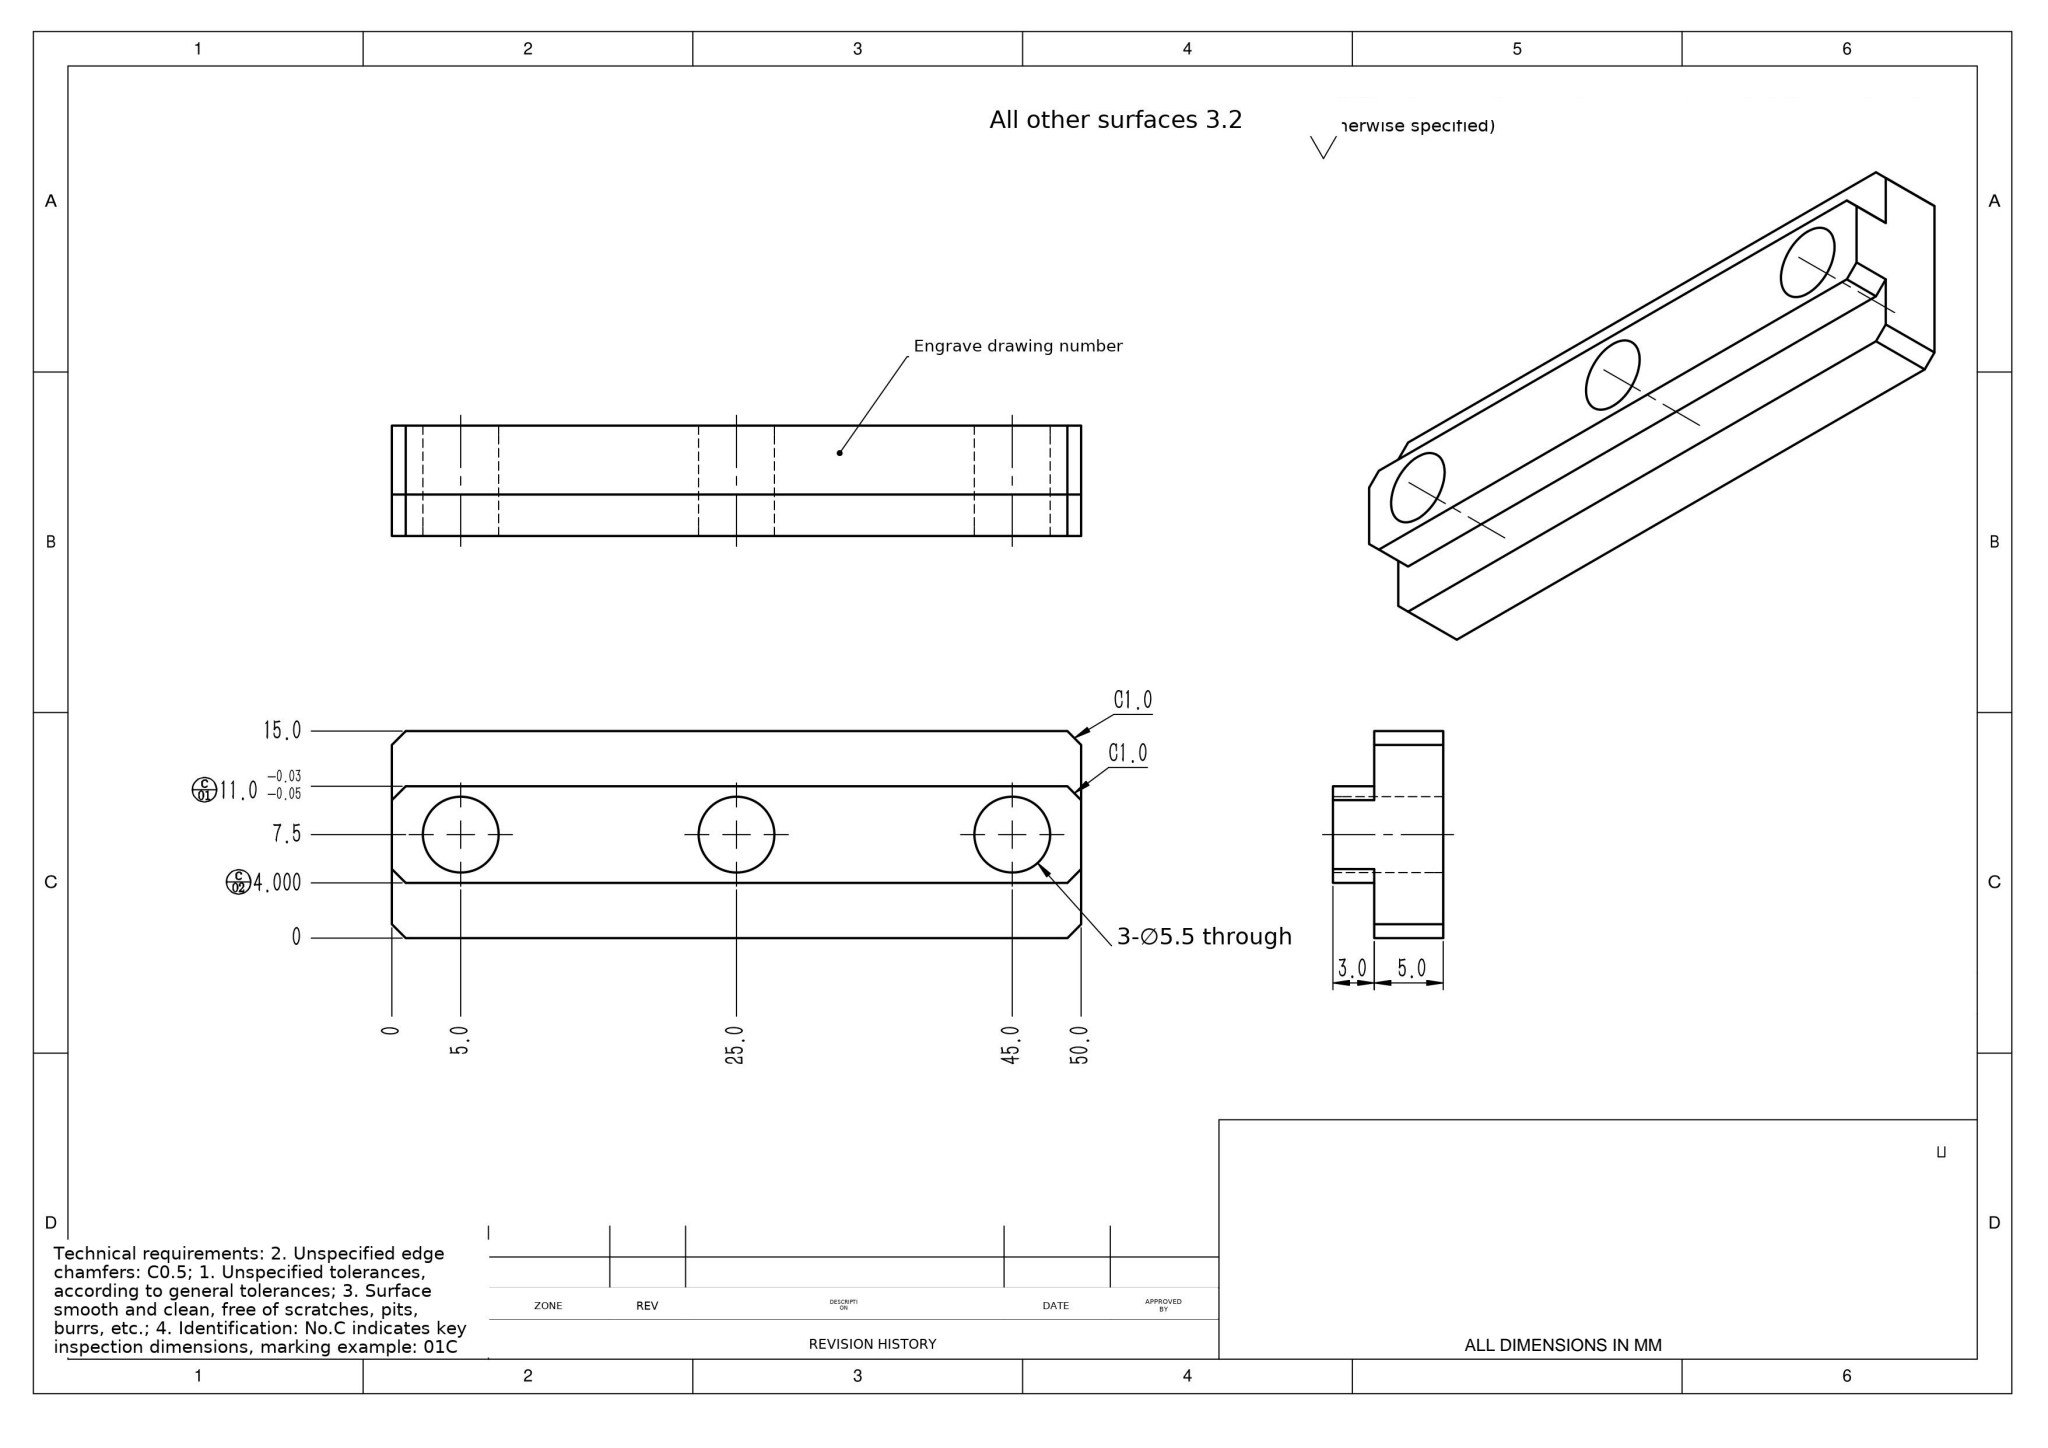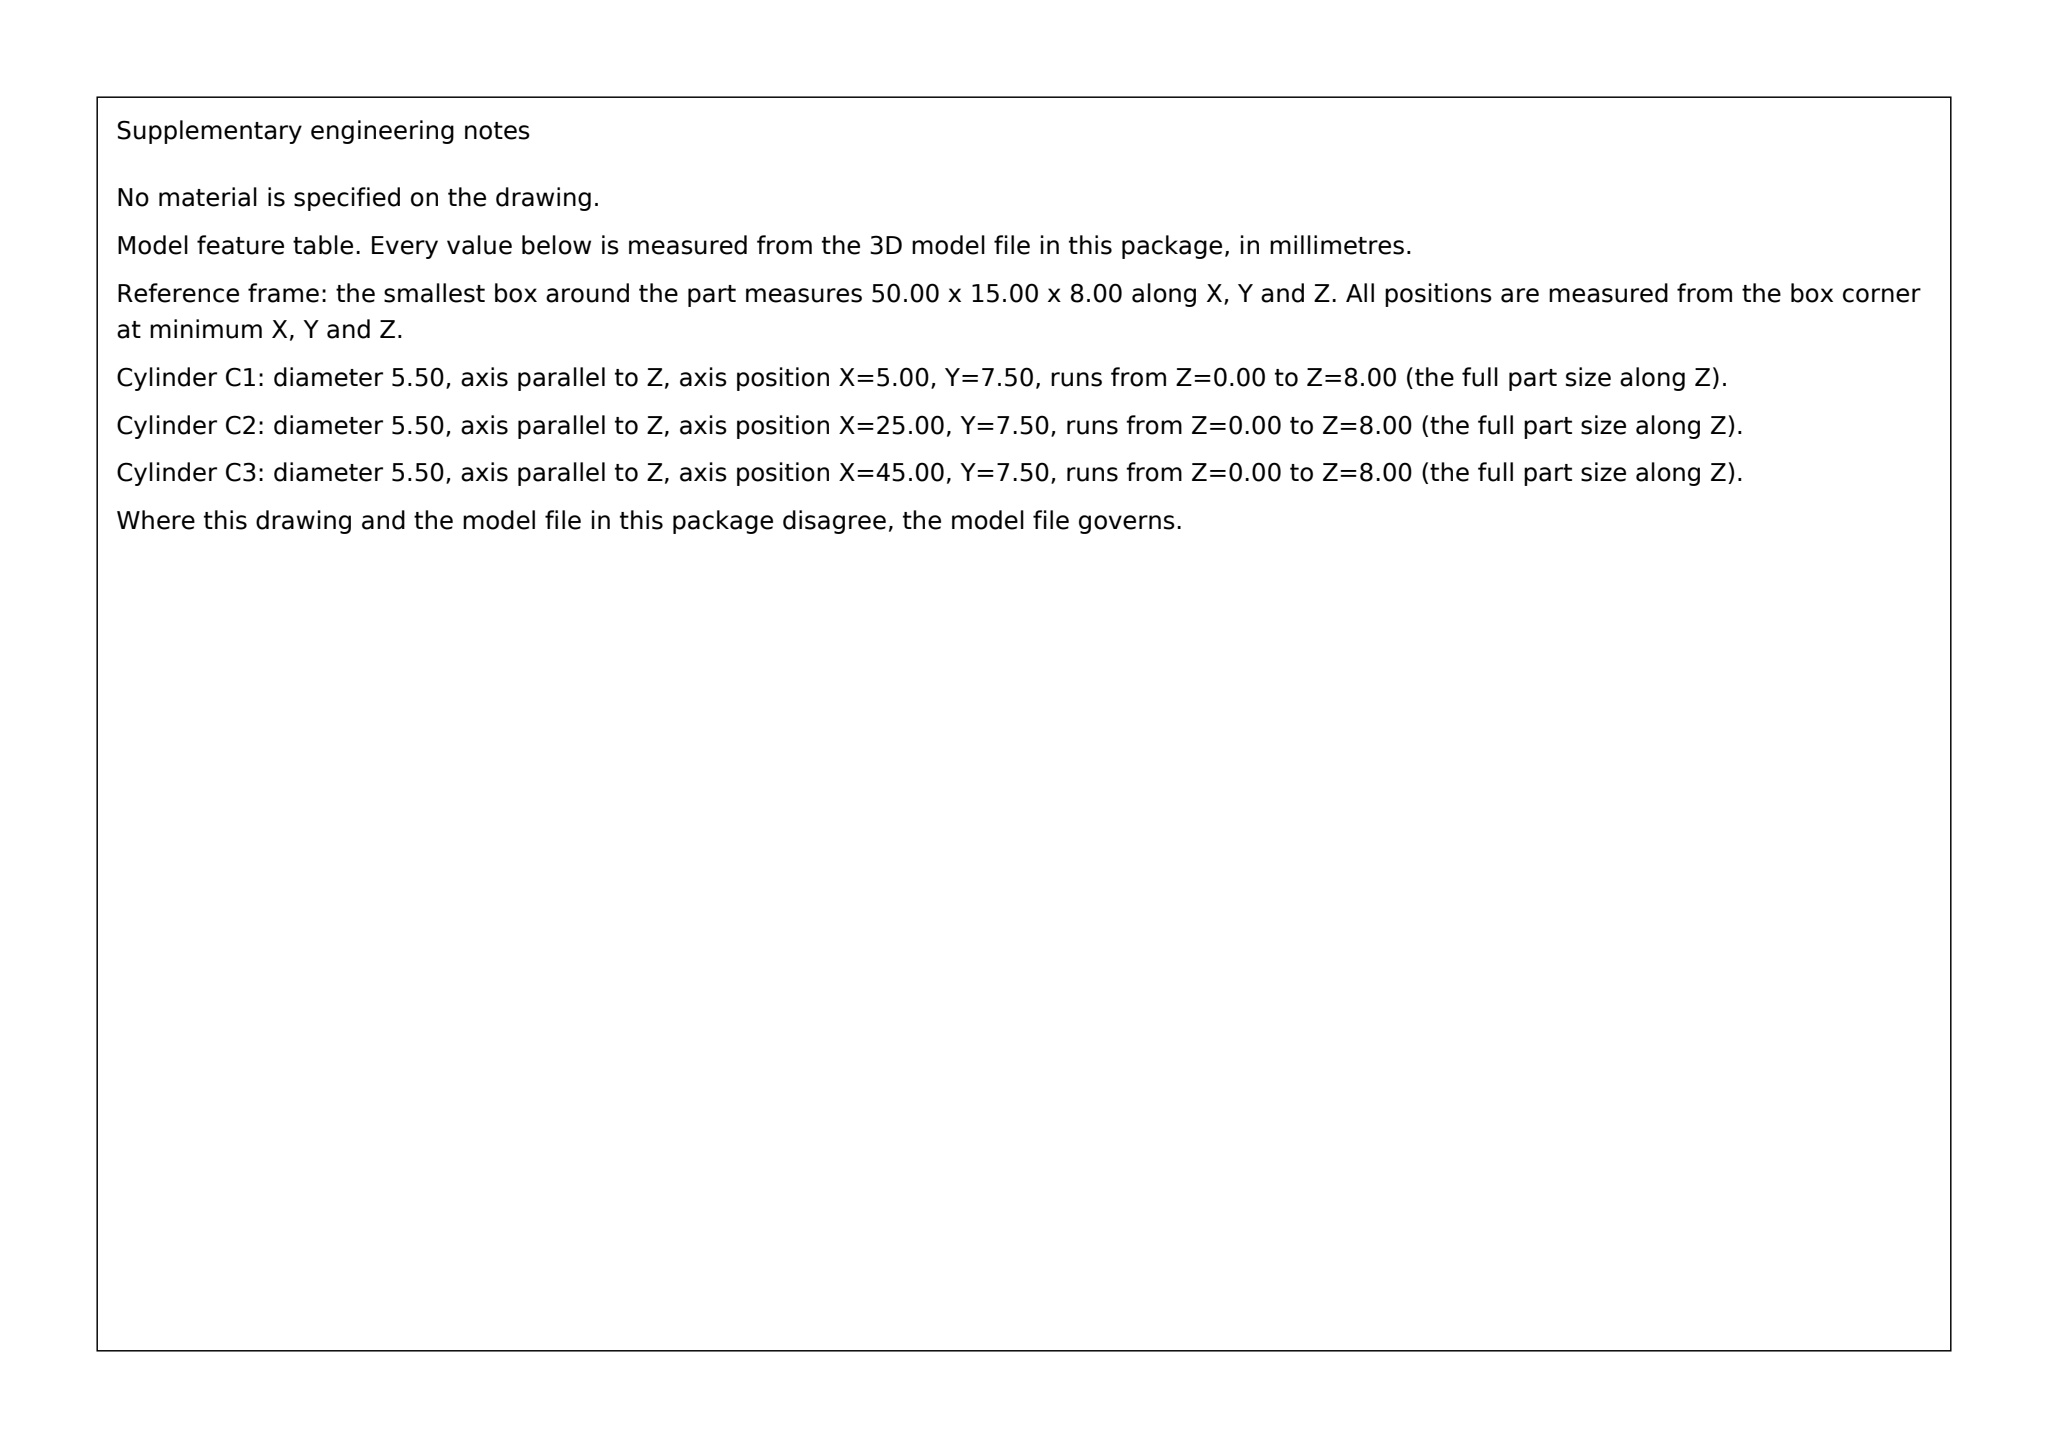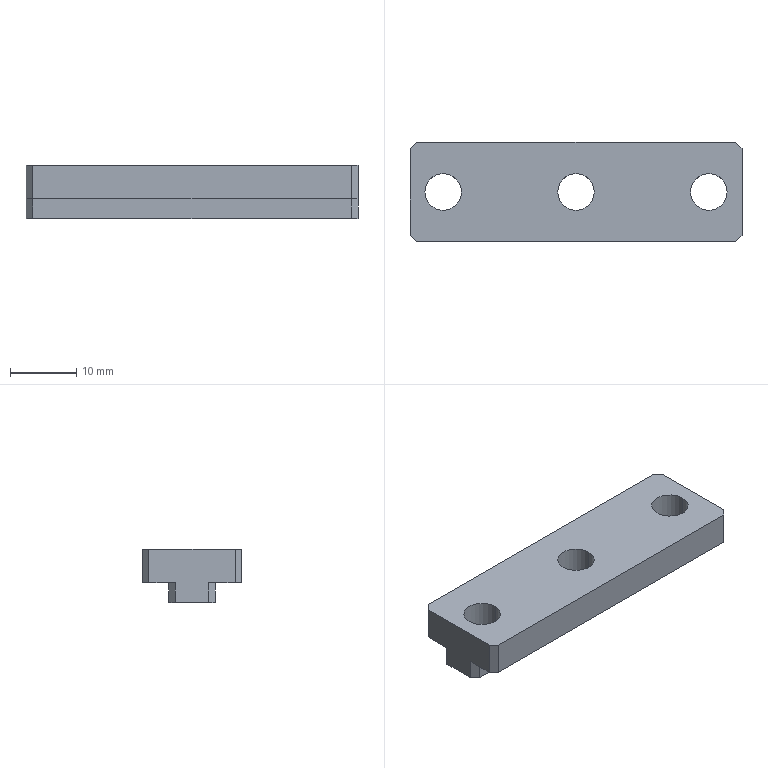Part | SolidWorks | mm | 1 solid | 24 faces | box 50 x 15 x 8 mm | volume 4214 mm3 | plane 18 | cylinder 6 | commonest cylinder face diameters 5.5 x6
build123d program:
from build123d import *

# Parameters (mm, degrees)
SKETCH2_W           = 50
SKETCH2_H           = 7
BOSS_EXTRUDE1_DEPTH = 3
SKETCH3_W           = 50
SKETCH3_H           = 15
BOSS_EXTRUDE2_DEPTH = 5
SKETCH4_R           = 2.75
CUT_EXTRUDE1_DEPTH  = 28.299
CHAMFER1_SIZE       = 1


with BuildPart() as part:
    # Sketch2 → Boss-Extrude1 (new body)
    with BuildSketch(Plane.XY):
        Rectangle(SKETCH2_W, SKETCH2_H)
    extrude(amount=BOSS_EXTRUDE1_DEPTH)

    # Sketch3 → Boss-Extrude2 (add)
    with BuildSketch(Plane.XY.offset(3)):
        Rectangle(SKETCH3_W, SKETCH3_H)
    extrude(amount=BOSS_EXTRUDE2_DEPTH)

    # Sketch4 → Cut-Extrude1 (cut, through all)
    with BuildSketch(Plane.XY.offset(8)):
        Circle(SKETCH4_R)
        with Locations((-20, 0)):
            Circle(SKETCH4_R)
        with Locations((20, 0)):
            Circle(SKETCH4_R)
    extrude(amount=-CUT_EXTRUDE1_DEPTH, mode=Mode.SUBTRACT)

    # Chamfer1
    chamfer1_edges = [part.edges().sort_by_distance(p)[0] for p in [
        (-25, -7.5, 5.5),
        (-25, -3.5, 1.5),
        (-25, 3.5, 1.5),
        (-25, 7.5, 5.5),
        (25, -7.5, 5.5),
        (25, -3.5, 1.5),
        (25, 3.5, 1.5),
        (25, 7.5, 5.5),
    ]]
    chamfer(chamfer1_edges, length=CHAMFER1_SIZE)


solid = part.part
STEP:
#1=CARTESIAN_POINT('',(22.75,0.,0.));
#2=VERTEX_POINT('',#1);
#3=CARTESIAN_POINT('',(17.25,0.,0.));
#4=VERTEX_POINT('',#3);
#5=CARTESIAN_POINT('',(20.,0.,0.));
#6=DIRECTION('',(0.,0.,-1.));
#7=DIRECTION('',(-1.,0.,0.));
#8=AXIS2_PLACEMENT_3D('',#5,#6,#7);
#9=CIRCLE('',#8,2.75);
#10=EDGE_CURVE('',#2,#4,#9,.T.);
#11=ORIENTED_EDGE('',*,*,#10,.T.);
#12=CARTESIAN_POINT('',(17.25,0.,8.));
#13=VERTEX_POINT('',#12);
#14=CARTESIAN_POINT('',(17.25,0.,-0.000025));
#15=DIRECTION('',(0.,0.,1.));
#16=VECTOR('',#15,1000.);
#17=LINE('',#14,#16);
#18=EDGE_CURVE('',#4,#13,#17,.T.);
#19=ORIENTED_EDGE('',*,*,#18,.T.);
#20=CARTESIAN_POINT('',(22.75,0.,8.));
#21=VERTEX_POINT('',#20);
#22=CARTESIAN_POINT('',(20.,0.,8.));
#23=DIRECTION('',(0.,0.,1.));
#24=DIRECTION('',(1.,0.,0.));
#25=AXIS2_PLACEMENT_3D('',#22,#23,#24);
#26=CIRCLE('',#25,2.75);
#27=EDGE_CURVE('',#13,#21,#26,.T.);
#28=ORIENTED_EDGE('',*,*,#27,.T.);
#29=CARTESIAN_POINT('',(22.75,0.,-0.000025));
#30=DIRECTION('',(0.,0.,1.));
#31=VECTOR('',#30,1000.);
#32=LINE('',#29,#31);
#33=EDGE_CURVE('',#2,#21,#32,.T.);
#34=ORIENTED_EDGE('',*,*,#33,.F.);
#35=EDGE_LOOP('',(#11,#19,#28,#34));
#36=FACE_OUTER_BOUND('',#35,.T.);
#37=CARTESIAN_POINT('',(20.,0.,-0.000025));
#38=DIRECTION('',(0.,0.,1.));
#39=DIRECTION('',(1.,0.,0.));
#40=AXIS2_PLACEMENT_3D('',#37,#38,#39);
#41=CYLINDRICAL_SURFACE('',#40,2.75);
#42=ADVANCED_FACE('',(#36),#41,.F.);
#43=CARTESIAN_POINT('',(-17.25,0.,0.));
#44=VERTEX_POINT('',#43);
#45=CARTESIAN_POINT('',(-22.75,0.,0.));
#46=VERTEX_POINT('',#45);
#47=CARTESIAN_POINT('',(-20.,0.,0.));
#48=DIRECTION('',(0.,0.,-1.));
#49=DIRECTION('',(-1.,0.,0.));
#50=AXIS2_PLACEMENT_3D('',#47,#48,#49);
#51=CIRCLE('',#50,2.75);
#52=EDGE_CURVE('',#44,#46,#51,.T.);
#53=ORIENTED_EDGE('',*,*,#52,.T.);
#54=CARTESIAN_POINT('',(-22.75,0.,8.));
#55=VERTEX_POINT('',#54);
#56=CARTESIAN_POINT('',(-22.75,0.,-0.000025));
#57=DIRECTION('',(0.,0.,1.));
#58=VECTOR('',#57,1000.);
#59=LINE('',#56,#58);
#60=EDGE_CURVE('',#46,#55,#59,.T.);
#61=ORIENTED_EDGE('',*,*,#60,.T.);
#62=CARTESIAN_POINT('',(-17.25,0.,8.));
#63=VERTEX_POINT('',#62);
#64=CARTESIAN_POINT('',(-20.,0.,8.));
#65=DIRECTION('',(0.,0.,1.));
#66=DIRECTION('',(1.,0.,0.));
#67=AXIS2_PLACEMENT_3D('',#64,#65,#66);
#68=CIRCLE('',#67,2.75);
#69=EDGE_CURVE('',#55,#63,#68,.T.);
#70=ORIENTED_EDGE('',*,*,#69,.T.);
#71=CARTESIAN_POINT('',(-17.25,0.,-0.000025));
#72=DIRECTION('',(0.,0.,1.));
#73=VECTOR('',#72,1000.);
#74=LINE('',#71,#73);
#75=EDGE_CURVE('',#44,#63,#74,.T.);
#76=ORIENTED_EDGE('',*,*,#75,.F.);
#77=EDGE_LOOP('',(#53,#61,#70,#76));
#78=FACE_OUTER_BOUND('',#77,.T.);
#79=CARTESIAN_POINT('',(-20.,0.,-0.000025));
#80=DIRECTION('',(0.,0.,1.));
#81=DIRECTION('',(1.,0.,0.));
#82=AXIS2_PLACEMENT_3D('',#79,#80,#81);
#83=CYLINDRICAL_SURFACE('',#82,2.75);
#84=ADVANCED_FACE('',(#78),#83,.F.);
#85=CARTESIAN_POINT('',(2.75,0.,0.));
#86=VERTEX_POINT('',#85);
#87=CARTESIAN_POINT('',(-2.75,0.,0.));
#88=VERTEX_POINT('',#87);
#89=CARTESIAN_POINT('',(0.,0.,0.));
#90=DIRECTION('',(0.,0.,-1.));
#91=DIRECTION('',(-1.,0.,0.));
#92=AXIS2_PLACEMENT_3D('',#89,#90,#91);
#93=CIRCLE('',#92,2.75);
#94=EDGE_CURVE('',#86,#88,#93,.T.);
#95=ORIENTED_EDGE('',*,*,#94,.T.);
#96=CARTESIAN_POINT('',(-2.75,0.,8.));
#97=VERTEX_POINT('',#96);
#98=CARTESIAN_POINT('',(-2.75,0.,-0.000025));
#99=DIRECTION('',(0.,0.,1.));
#100=VECTOR('',#99,1000.);
#101=LINE('',#98,#100);
#102=EDGE_CURVE('',#88,#97,#101,.T.);
#103=ORIENTED_EDGE('',*,*,#102,.T.);
#104=CARTESIAN_POINT('',(2.75,0.,8.));
#105=VERTEX_POINT('',#104);
#106=CARTESIAN_POINT('',(0.,0.,8.));
#107=DIRECTION('',(0.,0.,1.));
#108=DIRECTION('',(1.,0.,0.));
#109=AXIS2_PLACEMENT_3D('',#106,#107,#108);
#110=CIRCLE('',#109,2.75);
#111=EDGE_CURVE('',#97,#105,#110,.T.);
#112=ORIENTED_EDGE('',*,*,#111,.T.);
#113=CARTESIAN_POINT('',(2.75,0.,-0.000025));
#114=DIRECTION('',(0.,0.,1.));
#115=VECTOR('',#114,1000.);
#116=LINE('',#113,#115);
#117=EDGE_CURVE('',#86,#105,#116,.T.);
#118=ORIENTED_EDGE('',*,*,#117,.F.);
#119=EDGE_LOOP('',(#95,#103,#112,#118));
#120=FACE_OUTER_BOUND('',#119,.T.);
#121=CARTESIAN_POINT('',(0.,0.,-0.000025));
#122=DIRECTION('',(0.,0.,1.));
#123=DIRECTION('',(1.,0.,0.));
#124=AXIS2_PLACEMENT_3D('',#121,#122,#123);
#125=CYLINDRICAL_SURFACE('',#124,2.75);
#126=ADVANCED_FACE('',(#120),#125,.F.);
#127=CARTESIAN_POINT('',(25.,-6.5,8.));
#128=VERTEX_POINT('',#127);
#129=CARTESIAN_POINT('',(25.,6.5,8.));
#130=VERTEX_POINT('',#129);
#131=CARTESIAN_POINT('',(25.,-7.5,8.));
#132=DIRECTION('',(0.,1.,0.));
#133=VECTOR('',#132,1000.);
#134=LINE('',#131,#133);
#135=EDGE_CURVE('',#128,#130,#134,.T.);
#136=ORIENTED_EDGE('',*,*,#135,.F.);
#137=CARTESIAN_POINT('',(25.,-6.5,3.));
#138=VERTEX_POINT('',#137);
#139=CARTESIAN_POINT('',(25.,-6.5,3.));
#140=DIRECTION('',(0.,0.,-1.));
#141=VECTOR('',#140,1000.);
#142=LINE('',#139,#141);
#143=EDGE_CURVE('',#128,#138,#142,.T.);
#144=ORIENTED_EDGE('',*,*,#143,.T.);
#145=CARTESIAN_POINT('',(25.,-2.5,3.));
#146=VERTEX_POINT('',#145);
#147=CARTESIAN_POINT('',(25.,-7.5,3.));
#148=DIRECTION('',(0.,1.,0.));
#149=VECTOR('',#148,1000.);
#150=LINE('',#147,#149);
#151=EDGE_CURVE('',#138,#146,#150,.T.);
#152=ORIENTED_EDGE('',*,*,#151,.T.);
#153=CARTESIAN_POINT('',(25.,-2.5,0.));
#154=VERTEX_POINT('',#153);
#155=CARTESIAN_POINT('',(25.,-2.5,3.));
#156=DIRECTION('',(0.,0.,-1.));
#157=VECTOR('',#156,1000.);
#158=LINE('',#155,#157);
#159=EDGE_CURVE('',#146,#154,#158,.T.);
#160=ORIENTED_EDGE('',*,*,#159,.T.);
#161=CARTESIAN_POINT('',(25.,2.5,0.));
#162=VERTEX_POINT('',#161);
#163=CARTESIAN_POINT('',(25.,-3.5,0.));
#164=DIRECTION('',(0.,1.,0.));
#165=VECTOR('',#164,1000.);
#166=LINE('',#163,#165);
#167=EDGE_CURVE('',#154,#162,#166,.T.);
#168=ORIENTED_EDGE('',*,*,#167,.T.);
#169=CARTESIAN_POINT('',(25.,2.5,3.));
#170=VERTEX_POINT('',#169);
#171=CARTESIAN_POINT('',(25.,2.5,3.));
#172=DIRECTION('',(0.,0.,1.));
#173=VECTOR('',#172,1000.);
#174=LINE('',#171,#173);
#175=EDGE_CURVE('',#162,#170,#174,.T.);
#176=ORIENTED_EDGE('',*,*,#175,.T.);
#177=CARTESIAN_POINT('',(25.,6.5,3.));
#178=VERTEX_POINT('',#177);
#179=CARTESIAN_POINT('',(25.,-7.5,3.));
#180=DIRECTION('',(0.,1.,0.));
#181=VECTOR('',#180,1000.);
#182=LINE('',#179,#181);
#183=EDGE_CURVE('',#170,#178,#182,.T.);
#184=ORIENTED_EDGE('',*,*,#183,.T.);
#185=CARTESIAN_POINT('',(25.,6.5,3.));
#186=DIRECTION('',(0.,0.,1.));
#187=VECTOR('',#186,1000.);
#188=LINE('',#185,#187);
#189=EDGE_CURVE('',#178,#130,#188,.T.);
#190=ORIENTED_EDGE('',*,*,#189,.T.);
#191=EDGE_LOOP('',(#136,#144,#152,#160,#168,#176,#184,#190));
#192=FACE_OUTER_BOUND('',#191,.T.);
#193=CARTESIAN_POINT('',(25.,-3.5,3.));
#194=DIRECTION('',(-1.,0.,0.));
#195=DIRECTION('',(0.,0.,1.));
#196=AXIS2_PLACEMENT_3D('',#193,#194,#195);
#197=PLANE('',#196);
#198=ADVANCED_FACE('',(#192),#197,.F.);
#199=CARTESIAN_POINT('',(24.,3.5,0.));
#200=VERTEX_POINT('',#199);
#201=CARTESIAN_POINT('',(-24.,3.5,0.));
#202=VERTEX_POINT('',#201);
#203=CARTESIAN_POINT('',(-25.,3.5,0.));
#204=DIRECTION('',(-1.,0.,0.));
#205=VECTOR('',#204,1000.);
#206=LINE('',#203,#205);
#207=EDGE_CURVE('',#200,#202,#206,.T.);
#208=ORIENTED_EDGE('',*,*,#207,.T.);
#209=CARTESIAN_POINT('',(-24.,3.5,3.));
#210=VERTEX_POINT('',#209);
#211=CARTESIAN_POINT('',(-24.,3.5,3.));
#212=DIRECTION('',(0.,0.,1.));
#213=VECTOR('',#212,1000.);
#214=LINE('',#211,#213);
#215=EDGE_CURVE('',#202,#210,#214,.T.);
#216=ORIENTED_EDGE('',*,*,#215,.T.);
#217=CARTESIAN_POINT('',(24.,3.5,3.));
#218=VERTEX_POINT('',#217);
#219=CARTESIAN_POINT('',(-25.,3.5,3.));
#220=DIRECTION('',(-1.,0.,0.));
#221=VECTOR('',#220,1000.);
#222=LINE('',#219,#221);
#223=EDGE_CURVE('',#218,#210,#222,.T.);
#224=ORIENTED_EDGE('',*,*,#223,.F.);
#225=CARTESIAN_POINT('',(24.,3.5,3.));
#226=DIRECTION('',(0.,0.,-1.));
#227=VECTOR('',#226,1000.);
#228=LINE('',#225,#227);
#229=EDGE_CURVE('',#218,#200,#228,.T.);
#230=ORIENTED_EDGE('',*,*,#229,.T.);
#231=EDGE_LOOP('',(#208,#216,#224,#230));
#232=FACE_OUTER_BOUND('',#231,.T.);
#233=CARTESIAN_POINT('',(-25.,3.5,3.));
#234=DIRECTION('',(0.,-1.,0.));
#235=DIRECTION('',(0.,0.,-1.));
#236=AXIS2_PLACEMENT_3D('',#233,#234,#235);
#237=PLANE('',#236);
#238=ADVANCED_FACE('',(#232),#237,.F.);
#239=CARTESIAN_POINT('',(-25.,-2.5,3.));
#240=VERTEX_POINT('',#239);
#241=CARTESIAN_POINT('',(-25.,-6.5,3.));
#242=VERTEX_POINT('',#241);
#243=CARTESIAN_POINT('',(-25.,-7.5,3.));
#244=DIRECTION('',(0.,-1.,0.));
#245=VECTOR('',#244,1000.);
#246=LINE('',#243,#245);
#247=EDGE_CURVE('',#240,#242,#246,.T.);
#248=ORIENTED_EDGE('',*,*,#247,.T.);
#249=CARTESIAN_POINT('',(-25.,-6.5,8.));
#250=VERTEX_POINT('',#249);
#251=CARTESIAN_POINT('',(-25.,-6.5,3.));
#252=DIRECTION('',(0.,0.,1.));
#253=VECTOR('',#252,1000.);
#254=LINE('',#251,#253);
#255=EDGE_CURVE('',#242,#250,#254,.T.);
#256=ORIENTED_EDGE('',*,*,#255,.T.);
#257=CARTESIAN_POINT('',(-25.,6.5,8.));
#258=VERTEX_POINT('',#257);
#259=CARTESIAN_POINT('',(-25.,-7.5,8.));
#260=DIRECTION('',(0.,-1.,0.));
#261=VECTOR('',#260,1000.);
#262=LINE('',#259,#261);
#263=EDGE_CURVE('',#258,#250,#262,.T.);
#264=ORIENTED_EDGE('',*,*,#263,.F.);
#265=CARTESIAN_POINT('',(-25.,6.5,3.));
#266=VERTEX_POINT('',#265);
#267=CARTESIAN_POINT('',(-25.,6.5,3.));
#268=DIRECTION('',(0.,0.,-1.));
#269=VECTOR('',#268,1000.);
#270=LINE('',#267,#269);
#271=EDGE_CURVE('',#258,#266,#270,.T.);
#272=ORIENTED_EDGE('',*,*,#271,.T.);
#273=CARTESIAN_POINT('',(-25.,2.5,3.));
#274=VERTEX_POINT('',#273);
#275=CARTESIAN_POINT('',(-25.,-7.5,3.));
#276=DIRECTION('',(0.,-1.,0.));
#277=VECTOR('',#276,1000.);
#278=LINE('',#275,#277);
#279=EDGE_CURVE('',#266,#274,#278,.T.);
#280=ORIENTED_EDGE('',*,*,#279,.T.);
#281=CARTESIAN_POINT('',(-25.,2.5,0.));
#282=VERTEX_POINT('',#281);
#283=CARTESIAN_POINT('',(-25.,2.5,3.));
#284=DIRECTION('',(0.,0.,-1.));
#285=VECTOR('',#284,1000.);
#286=LINE('',#283,#285);
#287=EDGE_CURVE('',#274,#282,#286,.T.);
#288=ORIENTED_EDGE('',*,*,#287,.T.);
#289=CARTESIAN_POINT('',(-25.,-2.5,0.));
#290=VERTEX_POINT('',#289);
#291=CARTESIAN_POINT('',(-25.,-3.5,0.));
#292=DIRECTION('',(0.,-1.,0.));
#293=VECTOR('',#292,1000.);
#294=LINE('',#291,#293);
#295=EDGE_CURVE('',#282,#290,#294,.T.);
#296=ORIENTED_EDGE('',*,*,#295,.T.);
#297=CARTESIAN_POINT('',(-25.,-2.5,3.));
#298=DIRECTION('',(0.,0.,1.));
#299=VECTOR('',#298,1000.);
#300=LINE('',#297,#299);
#301=EDGE_CURVE('',#290,#240,#300,.T.);
#302=ORIENTED_EDGE('',*,*,#301,.T.);
#303=EDGE_LOOP('',(#248,#256,#264,#272,#280,#288,#296,#302));
#304=FACE_OUTER_BOUND('',#303,.T.);
#305=CARTESIAN_POINT('',(-25.,-3.5,3.));
#306=DIRECTION('',(1.,0.,0.));
#307=DIRECTION('',(0.,0.,-1.));
#308=AXIS2_PLACEMENT_3D('',#305,#306,#307);
#309=PLANE('',#308);
#310=ADVANCED_FACE('',(#304),#309,.F.);
#311=CARTESIAN_POINT('',(-24.,-3.5,3.));
#312=VERTEX_POINT('',#311);
#313=CARTESIAN_POINT('',(24.,-3.5,3.));
#314=VERTEX_POINT('',#313);
#315=CARTESIAN_POINT('',(-25.,-3.5,3.));
#316=DIRECTION('',(1.,0.,0.));
#317=VECTOR('',#316,1000.);
#318=LINE('',#315,#317);
#319=EDGE_CURVE('',#312,#314,#318,.T.);
#320=ORIENTED_EDGE('',*,*,#319,.F.);
#321=CARTESIAN_POINT('',(-24.,-3.5,0.));
#322=VERTEX_POINT('',#321);
#323=CARTESIAN_POINT('',(-24.,-3.5,3.));
#324=DIRECTION('',(0.,0.,-1.));
#325=VECTOR('',#324,1000.);
#326=LINE('',#323,#325);
#327=EDGE_CURVE('',#312,#322,#326,.T.);
#328=ORIENTED_EDGE('',*,*,#327,.T.);
#329=CARTESIAN_POINT('',(24.,-3.5,0.));
#330=VERTEX_POINT('',#329);
#331=CARTESIAN_POINT('',(-25.,-3.5,0.));
#332=DIRECTION('',(1.,0.,0.));
#333=VECTOR('',#332,1000.);
#334=LINE('',#331,#333);
#335=EDGE_CURVE('',#322,#330,#334,.T.);
#336=ORIENTED_EDGE('',*,*,#335,.T.);
#337=CARTESIAN_POINT('',(24.,-3.5,3.));
#338=DIRECTION('',(0.,0.,1.));
#339=VECTOR('',#338,1000.);
#340=LINE('',#337,#339);
#341=EDGE_CURVE('',#330,#314,#340,.T.);
#342=ORIENTED_EDGE('',*,*,#341,.T.);
#343=EDGE_LOOP('',(#320,#328,#336,#342));
#344=FACE_OUTER_BOUND('',#343,.T.);
#345=CARTESIAN_POINT('',(-25.,-3.5,3.));
#346=DIRECTION('',(0.,1.,0.));
#347=DIRECTION('',(0.,0.,1.));
#348=AXIS2_PLACEMENT_3D('',#345,#346,#347);
#349=PLANE('',#348);
#350=ADVANCED_FACE('',(#344),#349,.F.);
#351=ORIENTED_EDGE('',*,*,#10,.F.);
#352=CARTESIAN_POINT('',(20.,0.,0.));
#353=DIRECTION('',(0.,0.,-1.));
#354=DIRECTION('',(-1.,0.,0.));
#355=AXIS2_PLACEMENT_3D('',#352,#353,#354);
#356=CIRCLE('',#355,2.75);
#357=EDGE_CURVE('',#4,#2,#356,.T.);
#358=ORIENTED_EDGE('',*,*,#357,.F.);
#359=EDGE_LOOP('',(#351,#358));
#360=FACE_BOUND('',#359,.T.);
#361=ORIENTED_EDGE('',*,*,#52,.F.);
#362=CARTESIAN_POINT('',(-20.,0.,0.));
#363=DIRECTION('',(0.,0.,-1.));
#364=DIRECTION('',(-1.,0.,0.));
#365=AXIS2_PLACEMENT_3D('',#362,#363,#364);
#366=CIRCLE('',#365,2.75);
#367=EDGE_CURVE('',#46,#44,#366,.T.);
#368=ORIENTED_EDGE('',*,*,#367,.F.);
#369=EDGE_LOOP('',(#361,#368));
#370=FACE_BOUND('',#369,.T.);
#371=ORIENTED_EDGE('',*,*,#94,.F.);
#372=CARTESIAN_POINT('',(0.,0.,0.));
#373=DIRECTION('',(0.,0.,-1.));
#374=DIRECTION('',(-1.,0.,0.));
#375=AXIS2_PLACEMENT_3D('',#372,#373,#374);
#376=CIRCLE('',#375,2.75);
#377=EDGE_CURVE('',#88,#86,#376,.T.);
#378=ORIENTED_EDGE('',*,*,#377,.F.);
#379=EDGE_LOOP('',(#371,#378));
#380=FACE_BOUND('',#379,.T.);
#381=ORIENTED_EDGE('',*,*,#335,.F.);
#382=CARTESIAN_POINT('',(-13.75,-13.75,0.));
#383=DIRECTION('',(-0.7071,0.7071,0.));
#384=VECTOR('',#383,1000.);
#385=LINE('',#382,#384);
#386=EDGE_CURVE('',#322,#290,#385,.T.);
#387=ORIENTED_EDGE('',*,*,#386,.T.);
#388=ORIENTED_EDGE('',*,*,#295,.F.);
#389=CARTESIAN_POINT('',(-13.75,13.75,0.));
#390=DIRECTION('',(0.7071,0.7071,0.));
#391=VECTOR('',#390,1000.);
#392=LINE('',#389,#391);
#393=EDGE_CURVE('',#282,#202,#392,.T.);
#394=ORIENTED_EDGE('',*,*,#393,.T.);
#395=ORIENTED_EDGE('',*,*,#207,.F.);
#396=CARTESIAN_POINT('',(13.75,13.75,0.));
#397=DIRECTION('',(0.7071,-0.7071,0.));
#398=VECTOR('',#397,1000.);
#399=LINE('',#396,#398);
#400=EDGE_CURVE('',#200,#162,#399,.T.);
#401=ORIENTED_EDGE('',*,*,#400,.T.);
#402=ORIENTED_EDGE('',*,*,#167,.F.);
#403=CARTESIAN_POINT('',(13.75,-13.75,0.));
#404=DIRECTION('',(-0.7071,-0.7071,0.));
#405=VECTOR('',#404,1000.);
#406=LINE('',#403,#405);
#407=EDGE_CURVE('',#154,#330,#406,.T.);
#408=ORIENTED_EDGE('',*,*,#407,.T.);
#409=EDGE_LOOP('',(#381,#387,#388,#394,#395,#401,#402,#408));
#410=FACE_OUTER_BOUND('',#409,.T.);
#411=CARTESIAN_POINT('',(0.,0.,0.));
#412=DIRECTION('',(0.,0.,-1.));
#413=DIRECTION('',(-1.,0.,0.));
#414=AXIS2_PLACEMENT_3D('',#411,#412,#413);
#415=PLANE('',#414);
#416=ADVANCED_FACE('',(#360,#370,#380,#410),#415,.T.);
#417=ORIENTED_EDGE('',*,*,#279,.F.);
#418=CARTESIAN_POINT('',(-24.,7.5,3.));
#419=VERTEX_POINT('',#418);
#420=CARTESIAN_POINT('',(-15.75,15.75,3.));
#421=DIRECTION('',(0.7071,0.7071,0.));
#422=VECTOR('',#421,1000.);
#423=LINE('',#420,#422);
#424=EDGE_CURVE('',#266,#419,#423,.T.);
#425=ORIENTED_EDGE('',*,*,#424,.T.);
#426=CARTESIAN_POINT('',(24.,7.5,3.));
#427=VERTEX_POINT('',#426);
#428=CARTESIAN_POINT('',(-25.,7.5,3.));
#429=DIRECTION('',(-1.,0.,0.));
#430=VECTOR('',#429,1000.);
#431=LINE('',#428,#430);
#432=EDGE_CURVE('',#427,#419,#431,.T.);
#433=ORIENTED_EDGE('',*,*,#432,.F.);
#434=CARTESIAN_POINT('',(15.75,15.75,3.));
#435=DIRECTION('',(0.7071,-0.7071,0.));
#436=VECTOR('',#435,1000.);
#437=LINE('',#434,#436);
#438=EDGE_CURVE('',#427,#178,#437,.T.);
#439=ORIENTED_EDGE('',*,*,#438,.T.);
#440=ORIENTED_EDGE('',*,*,#183,.F.);
#441=CARTESIAN_POINT('',(24.,3.5,3.));
#442=DIRECTION('',(-0.7071,0.7071,0.));
#443=VECTOR('',#442,1000.);
#444=LINE('',#441,#443);
#445=EDGE_CURVE('',#170,#218,#444,.T.);
#446=ORIENTED_EDGE('',*,*,#445,.T.);
#447=ORIENTED_EDGE('',*,*,#223,.T.);
#448=CARTESIAN_POINT('',(-25.,2.5,3.));
#449=DIRECTION('',(-0.7071,-0.7071,0.));
#450=VECTOR('',#449,1000.);
#451=LINE('',#448,#450);
#452=EDGE_CURVE('',#210,#274,#451,.T.);
#453=ORIENTED_EDGE('',*,*,#452,.T.);
#454=EDGE_LOOP('',(#417,#425,#433,#439,#440,#446,#447,#453));
#455=FACE_OUTER_BOUND('',#454,.T.);
#456=CARTESIAN_POINT('',(0.,0.,3.));
#457=DIRECTION('',(0.,0.,-1.));
#458=DIRECTION('',(-1.,0.,0.));
#459=AXIS2_PLACEMENT_3D('',#456,#457,#458);
#460=PLANE('',#459);
#461=ADVANCED_FACE('',(#455),#460,.T.);
#462=ORIENTED_EDGE('',*,*,#432,.T.);
#463=CARTESIAN_POINT('',(-24.,7.5,8.));
#464=VERTEX_POINT('',#463);
#465=CARTESIAN_POINT('',(-24.,7.5,8.));
#466=DIRECTION('',(0.,0.,1.));
#467=VECTOR('',#466,1000.);
#468=LINE('',#465,#467);
#469=EDGE_CURVE('',#419,#464,#468,.T.);
#470=ORIENTED_EDGE('',*,*,#469,.T.);
#471=CARTESIAN_POINT('',(24.,7.5,8.));
#472=VERTEX_POINT('',#471);
#473=CARTESIAN_POINT('',(-25.,7.5,8.));
#474=DIRECTION('',(-1.,0.,0.));
#475=VECTOR('',#474,1000.);
#476=LINE('',#473,#475);
#477=EDGE_CURVE('',#472,#464,#476,.T.);
#478=ORIENTED_EDGE('',*,*,#477,.F.);
#479=CARTESIAN_POINT('',(24.,7.5,8.));
#480=DIRECTION('',(0.,0.,-1.));
#481=VECTOR('',#480,1000.);
#482=LINE('',#479,#481);
#483=EDGE_CURVE('',#472,#427,#482,.T.);
#484=ORIENTED_EDGE('',*,*,#483,.T.);
#485=EDGE_LOOP('',(#462,#470,#478,#484));
#486=FACE_OUTER_BOUND('',#485,.T.);
#487=CARTESIAN_POINT('',(-25.,7.5,8.));
#488=DIRECTION('',(0.,-1.,0.));
#489=DIRECTION('',(0.,0.,-1.));
#490=AXIS2_PLACEMENT_3D('',#487,#488,#489);
#491=PLANE('',#490);
#492=ADVANCED_FACE('',(#486),#491,.F.);
#493=CARTESIAN_POINT('',(-24.,-7.5,8.));
#494=VERTEX_POINT('',#493);
#495=CARTESIAN_POINT('',(24.,-7.5,8.));
#496=VERTEX_POINT('',#495);
#497=CARTESIAN_POINT('',(-25.,-7.5,8.));
#498=DIRECTION('',(1.,0.,0.));
#499=VECTOR('',#498,1000.);
#500=LINE('',#497,#499);
#501=EDGE_CURVE('',#494,#496,#500,.T.);
#502=ORIENTED_EDGE('',*,*,#501,.F.);
#503=CARTESIAN_POINT('',(-24.,-7.5,3.));
#504=VERTEX_POINT('',#503);
#505=CARTESIAN_POINT('',(-24.,-7.5,8.));
#506=DIRECTION('',(0.,0.,-1.));
#507=VECTOR('',#506,1000.);
#508=LINE('',#505,#507);
#509=EDGE_CURVE('',#494,#504,#508,.T.);
#510=ORIENTED_EDGE('',*,*,#509,.T.);
#511=CARTESIAN_POINT('',(24.,-7.5,3.));
#512=VERTEX_POINT('',#511);
#513=CARTESIAN_POINT('',(-25.,-7.5,3.));
#514=DIRECTION('',(1.,0.,0.));
#515=VECTOR('',#514,1000.);
#516=LINE('',#513,#515);
#517=EDGE_CURVE('',#504,#512,#516,.T.);
#518=ORIENTED_EDGE('',*,*,#517,.T.);
#519=CARTESIAN_POINT('',(24.,-7.5,8.));
#520=DIRECTION('',(0.,0.,1.));
#521=VECTOR('',#520,1000.);
#522=LINE('',#519,#521);
#523=EDGE_CURVE('',#512,#496,#522,.T.);
#524=ORIENTED_EDGE('',*,*,#523,.T.);
#525=EDGE_LOOP('',(#502,#510,#518,#524));
#526=FACE_OUTER_BOUND('',#525,.T.);
#527=CARTESIAN_POINT('',(-25.,-7.5,8.));
#528=DIRECTION('',(0.,1.,0.));
#529=DIRECTION('',(0.,0.,1.));
#530=AXIS2_PLACEMENT_3D('',#527,#528,#529);
#531=PLANE('',#530);
#532=ADVANCED_FACE('',(#526),#531,.F.);
#533=CARTESIAN_POINT('',(20.,0.,8.));
#534=DIRECTION('',(0.,0.,1.));
#535=DIRECTION('',(1.,0.,0.));
#536=AXIS2_PLACEMENT_3D('',#533,#534,#535);
#537=CIRCLE('',#536,2.75);
#538=EDGE_CURVE('',#21,#13,#537,.T.);
#539=ORIENTED_EDGE('',*,*,#538,.F.);
#540=ORIENTED_EDGE('',*,*,#27,.F.);
#541=EDGE_LOOP('',(#539,#540));
#542=FACE_BOUND('',#541,.T.);
#543=CARTESIAN_POINT('',(-20.,0.,8.));
#544=DIRECTION('',(0.,0.,1.));
#545=DIRECTION('',(1.,0.,0.));
#546=AXIS2_PLACEMENT_3D('',#543,#544,#545);
#547=CIRCLE('',#546,2.75);
#548=EDGE_CURVE('',#63,#55,#547,.T.);
#549=ORIENTED_EDGE('',*,*,#548,.F.);
#550=ORIENTED_EDGE('',*,*,#69,.F.);
#551=EDGE_LOOP('',(#549,#550));
#552=FACE_BOUND('',#551,.T.);
#553=CARTESIAN_POINT('',(0.,0.,8.));
#554=DIRECTION('',(0.,0.,1.));
#555=DIRECTION('',(1.,0.,0.));
#556=AXIS2_PLACEMENT_3D('',#553,#554,#555);
#557=CIRCLE('',#556,2.75);
#558=EDGE_CURVE('',#105,#97,#557,.T.);
#559=ORIENTED_EDGE('',*,*,#558,.F.);
#560=ORIENTED_EDGE('',*,*,#111,.F.);
#561=EDGE_LOOP('',(#559,#560));
#562=FACE_BOUND('',#561,.T.);
#563=ORIENTED_EDGE('',*,*,#263,.T.);
#564=CARTESIAN_POINT('',(-24.,-7.5,8.));
#565=DIRECTION('',(0.7071,-0.7071,0.));
#566=VECTOR('',#565,1000.);
#567=LINE('',#564,#566);
#568=EDGE_CURVE('',#250,#494,#567,.T.);
#569=ORIENTED_EDGE('',*,*,#568,.T.);
#570=ORIENTED_EDGE('',*,*,#501,.T.);
#571=CARTESIAN_POINT('',(25.,-6.5,8.));
#572=DIRECTION('',(0.7071,0.7071,0.));
#573=VECTOR('',#572,1000.);
#574=LINE('',#571,#573);
#575=EDGE_CURVE('',#496,#128,#574,.T.);
#576=ORIENTED_EDGE('',*,*,#575,.T.);
#577=ORIENTED_EDGE('',*,*,#135,.T.);
#578=CARTESIAN_POINT('',(24.,7.5,8.));
#579=DIRECTION('',(-0.7071,0.7071,0.));
#580=VECTOR('',#579,1000.);
#581=LINE('',#578,#580);
#582=EDGE_CURVE('',#130,#472,#581,.T.);
#583=ORIENTED_EDGE('',*,*,#582,.T.);
#584=ORIENTED_EDGE('',*,*,#477,.T.);
#585=CARTESIAN_POINT('',(-25.,6.5,8.));
#586=DIRECTION('',(-0.7071,-0.7071,0.));
#587=VECTOR('',#586,1000.);
#588=LINE('',#585,#587);
#589=EDGE_CURVE('',#464,#258,#588,.T.);
#590=ORIENTED_EDGE('',*,*,#589,.T.);
#591=EDGE_LOOP('',(#563,#569,#570,#576,#577,#583,#584,#590));
#592=FACE_OUTER_BOUND('',#591,.T.);
#593=CARTESIAN_POINT('',(0.,0.,8.));
#594=DIRECTION('',(0.,0.,-1.));
#595=DIRECTION('',(-1.,0.,0.));
#596=AXIS2_PLACEMENT_3D('',#593,#594,#595);
#597=PLANE('',#596);
#598=ADVANCED_FACE('',(#542,#552,#562,#592),#597,.F.);
#599=ORIENTED_EDGE('',*,*,#517,.F.);
#600=CARTESIAN_POINT('',(-15.75,-15.75,3.));
#601=DIRECTION('',(-0.7071,0.7071,0.));
#602=VECTOR('',#601,1000.);
#603=LINE('',#600,#602);
#604=EDGE_CURVE('',#504,#242,#603,.T.);
#605=ORIENTED_EDGE('',*,*,#604,.T.);
#606=ORIENTED_EDGE('',*,*,#247,.F.);
#607=CARTESIAN_POINT('',(-24.,-3.5,3.));
#608=DIRECTION('',(0.7071,-0.7071,0.));
#609=VECTOR('',#608,1000.);
#610=LINE('',#607,#609);
#611=EDGE_CURVE('',#240,#312,#610,.T.);
#612=ORIENTED_EDGE('',*,*,#611,.T.);
#613=ORIENTED_EDGE('',*,*,#319,.T.);
#614=CARTESIAN_POINT('',(25.,-2.5,3.));
#615=DIRECTION('',(0.7071,0.7071,0.));
#616=VECTOR('',#615,1000.);
#617=LINE('',#614,#616);
#618=EDGE_CURVE('',#314,#146,#617,.T.);
#619=ORIENTED_EDGE('',*,*,#618,.T.);
#620=ORIENTED_EDGE('',*,*,#151,.F.);
#621=CARTESIAN_POINT('',(15.75,-15.75,3.));
#622=DIRECTION('',(-0.7071,-0.7071,0.));
#623=VECTOR('',#622,1000.);
#624=LINE('',#621,#623);
#625=EDGE_CURVE('',#138,#512,#624,.T.);
#626=ORIENTED_EDGE('',*,*,#625,.T.);
#627=EDGE_LOOP('',(#599,#605,#606,#612,#613,#619,#620,#626));
#628=FACE_OUTER_BOUND('',#627,.T.);
#629=CARTESIAN_POINT('',(0.,0.,3.));
#630=DIRECTION('',(0.,0.,-1.));
#631=DIRECTION('',(-1.,0.,0.));
#632=AXIS2_PLACEMENT_3D('',#629,#630,#631);
#633=PLANE('',#632);
#634=ADVANCED_FACE('',(#628),#633,.T.);
#635=ORIENTED_EDGE('',*,*,#102,.F.);
#636=ORIENTED_EDGE('',*,*,#377,.T.);
#637=ORIENTED_EDGE('',*,*,#117,.T.);
#638=ORIENTED_EDGE('',*,*,#558,.T.);
#639=EDGE_LOOP('',(#635,#636,#637,#638));
#640=FACE_OUTER_BOUND('',#639,.T.);
#641=CARTESIAN_POINT('',(0.,0.,-0.000025));
#642=DIRECTION('',(0.,0.,1.));
#643=DIRECTION('',(1.,0.,0.));
#644=AXIS2_PLACEMENT_3D('',#641,#642,#643);
#645=CYLINDRICAL_SURFACE('',#644,2.75);
#646=ADVANCED_FACE('',(#640),#645,.F.);
#647=ORIENTED_EDGE('',*,*,#60,.F.);
#648=ORIENTED_EDGE('',*,*,#367,.T.);
#649=ORIENTED_EDGE('',*,*,#75,.T.);
#650=ORIENTED_EDGE('',*,*,#548,.T.);
#651=EDGE_LOOP('',(#647,#648,#649,#650));
#652=FACE_OUTER_BOUND('',#651,.T.);
#653=CARTESIAN_POINT('',(-20.,0.,-0.000025));
#654=DIRECTION('',(0.,0.,1.));
#655=DIRECTION('',(1.,0.,0.));
#656=AXIS2_PLACEMENT_3D('',#653,#654,#655);
#657=CYLINDRICAL_SURFACE('',#656,2.75);
#658=ADVANCED_FACE('',(#652),#657,.F.);
#659=ORIENTED_EDGE('',*,*,#18,.F.);
#660=ORIENTED_EDGE('',*,*,#357,.T.);
#661=ORIENTED_EDGE('',*,*,#33,.T.);
#662=ORIENTED_EDGE('',*,*,#538,.T.);
#663=EDGE_LOOP('',(#659,#660,#661,#662));
#664=FACE_OUTER_BOUND('',#663,.T.);
#665=CARTESIAN_POINT('',(20.,0.,-0.000025));
#666=DIRECTION('',(0.,0.,1.));
#667=DIRECTION('',(1.,0.,0.));
#668=AXIS2_PLACEMENT_3D('',#665,#666,#667);
#669=CYLINDRICAL_SURFACE('',#668,2.75);
#670=ADVANCED_FACE('',(#664),#669,.F.);
#671=ORIENTED_EDGE('',*,*,#568,.F.);
#672=ORIENTED_EDGE('',*,*,#255,.F.);
#673=ORIENTED_EDGE('',*,*,#604,.F.);
#674=ORIENTED_EDGE('',*,*,#509,.F.);
#675=EDGE_LOOP('',(#671,#672,#673,#674));
#676=FACE_OUTER_BOUND('',#675,.T.);
#677=CARTESIAN_POINT('',(-24.,-7.5,8.));
#678=DIRECTION('',(0.7071,0.7071,0.));
#679=DIRECTION('',(0.,0.,-1.));
#680=AXIS2_PLACEMENT_3D('',#677,#678,#679);
#681=PLANE('',#680);
#682=ADVANCED_FACE('',(#676),#681,.F.);
#683=ORIENTED_EDGE('',*,*,#611,.F.);
#684=ORIENTED_EDGE('',*,*,#301,.F.);
#685=ORIENTED_EDGE('',*,*,#386,.F.);
#686=ORIENTED_EDGE('',*,*,#327,.F.);
#687=EDGE_LOOP('',(#683,#684,#685,#686));
#688=FACE_OUTER_BOUND('',#687,.T.);
#689=CARTESIAN_POINT('',(-24.,-3.5,3.));
#690=DIRECTION('',(0.7071,0.7071,0.));
#691=DIRECTION('',(0.,0.,-1.));
#692=AXIS2_PLACEMENT_3D('',#689,#690,#691);
#693=PLANE('',#692);
#694=ADVANCED_FACE('',(#688),#693,.F.);
#695=ORIENTED_EDGE('',*,*,#452,.F.);
#696=ORIENTED_EDGE('',*,*,#215,.F.);
#697=ORIENTED_EDGE('',*,*,#393,.F.);
#698=ORIENTED_EDGE('',*,*,#287,.F.);
#699=EDGE_LOOP('',(#695,#696,#697,#698));
#700=FACE_OUTER_BOUND('',#699,.T.);
#701=CARTESIAN_POINT('',(-25.,2.5,3.));
#702=DIRECTION('',(0.7071,-0.7071,0.));
#703=DIRECTION('',(0.,0.,-1.));
#704=AXIS2_PLACEMENT_3D('',#701,#702,#703);
#705=PLANE('',#704);
#706=ADVANCED_FACE('',(#700),#705,.F.);
#707=ORIENTED_EDGE('',*,*,#589,.F.);
#708=ORIENTED_EDGE('',*,*,#469,.F.);
#709=ORIENTED_EDGE('',*,*,#424,.F.);
#710=ORIENTED_EDGE('',*,*,#271,.F.);
#711=EDGE_LOOP('',(#707,#708,#709,#710));
#712=FACE_OUTER_BOUND('',#711,.T.);
#713=CARTESIAN_POINT('',(-25.,6.5,3.));
#714=DIRECTION('',(0.7071,-0.7071,0.));
#715=DIRECTION('',(0.,0.,-1.));
#716=AXIS2_PLACEMENT_3D('',#713,#714,#715);
#717=PLANE('',#716);
#718=ADVANCED_FACE('',(#712),#717,.F.);
#719=ORIENTED_EDGE('',*,*,#575,.F.);
#720=ORIENTED_EDGE('',*,*,#523,.F.);
#721=ORIENTED_EDGE('',*,*,#625,.F.);
#722=ORIENTED_EDGE('',*,*,#143,.F.);
#723=EDGE_LOOP('',(#719,#720,#721,#722));
#724=FACE_OUTER_BOUND('',#723,.T.);
#725=CARTESIAN_POINT('',(25.,-6.5,3.));
#726=DIRECTION('',(-0.7071,0.7071,0.));
#727=DIRECTION('',(0.,0.,-1.));
#728=AXIS2_PLACEMENT_3D('',#725,#726,#727);
#729=PLANE('',#728);
#730=ADVANCED_FACE('',(#724),#729,.F.);
#731=ORIENTED_EDGE('',*,*,#618,.F.);
#732=ORIENTED_EDGE('',*,*,#341,.F.);
#733=ORIENTED_EDGE('',*,*,#407,.F.);
#734=ORIENTED_EDGE('',*,*,#159,.F.);
#735=EDGE_LOOP('',(#731,#732,#733,#734));
#736=FACE_OUTER_BOUND('',#735,.T.);
#737=CARTESIAN_POINT('',(25.,-2.5,3.));
#738=DIRECTION('',(-0.7071,0.7071,0.));
#739=DIRECTION('',(0.,0.,-1.));
#740=AXIS2_PLACEMENT_3D('',#737,#738,#739);
#741=PLANE('',#740);
#742=ADVANCED_FACE('',(#736),#741,.F.);
#743=ORIENTED_EDGE('',*,*,#445,.F.);
#744=ORIENTED_EDGE('',*,*,#175,.F.);
#745=ORIENTED_EDGE('',*,*,#400,.F.);
#746=ORIENTED_EDGE('',*,*,#229,.F.);
#747=EDGE_LOOP('',(#743,#744,#745,#746));
#748=FACE_OUTER_BOUND('',#747,.T.);
#749=CARTESIAN_POINT('',(24.,3.5,3.));
#750=DIRECTION('',(-0.7071,-0.7071,0.));
#751=DIRECTION('',(0.,0.,-1.));
#752=AXIS2_PLACEMENT_3D('',#749,#750,#751);
#753=PLANE('',#752);
#754=ADVANCED_FACE('',(#748),#753,.F.);
#755=ORIENTED_EDGE('',*,*,#582,.F.);
#756=ORIENTED_EDGE('',*,*,#189,.F.);
#757=ORIENTED_EDGE('',*,*,#438,.F.);
#758=ORIENTED_EDGE('',*,*,#483,.F.);
#759=EDGE_LOOP('',(#755,#756,#757,#758));
#760=FACE_OUTER_BOUND('',#759,.T.);
#761=CARTESIAN_POINT('',(24.,7.5,8.));
#762=DIRECTION('',(-0.7071,-0.7071,0.));
#763=DIRECTION('',(0.,0.,-1.));
#764=AXIS2_PLACEMENT_3D('',#761,#762,#763);
#765=PLANE('',#764);
#766=ADVANCED_FACE('',(#760),#765,.F.);
#767=CLOSED_SHELL('',(#42,#84,#126,#198,#238,#310,#350,#416,#461,#492,#532,#598,#634,#646,#658,#670,#682,#694,#706,#718,#730,#742,#754,#766));
#768=MANIFOLD_SOLID_BREP('',#767);
#769=CARTESIAN_POINT('',(0.,0.,0.));
#770=DIRECTION('',(0.,0.,1.));
#771=DIRECTION('',(1.,0.,0.));
#772=AXIS2_PLACEMENT_3D('',#769,#770,#771);
#773=(LENGTH_UNIT()NAMED_UNIT(*)SI_UNIT(.MILLI.,.METRE.));
#774=UNCERTAINTY_MEASURE_WITH_UNIT(LENGTH_MEASURE(0.00001),#773,'','');
#775=(NAMED_UNIT(*)PLANE_ANGLE_UNIT()SI_UNIT($,.RADIAN.));
#776=(NAMED_UNIT(*)SI_UNIT($,.STERADIAN.)SOLID_ANGLE_UNIT());
#777=(GEOMETRIC_REPRESENTATION_CONTEXT(3)GLOBAL_UNCERTAINTY_ASSIGNED_CONTEXT((#774))GLOBAL_UNIT_ASSIGNED_CONTEXT((#773,#775,#776))REPRESENTATION_CONTEXT('',''));
#778=ADVANCED_BREP_SHAPE_REPRESENTATION('',(#768,#772),#777);